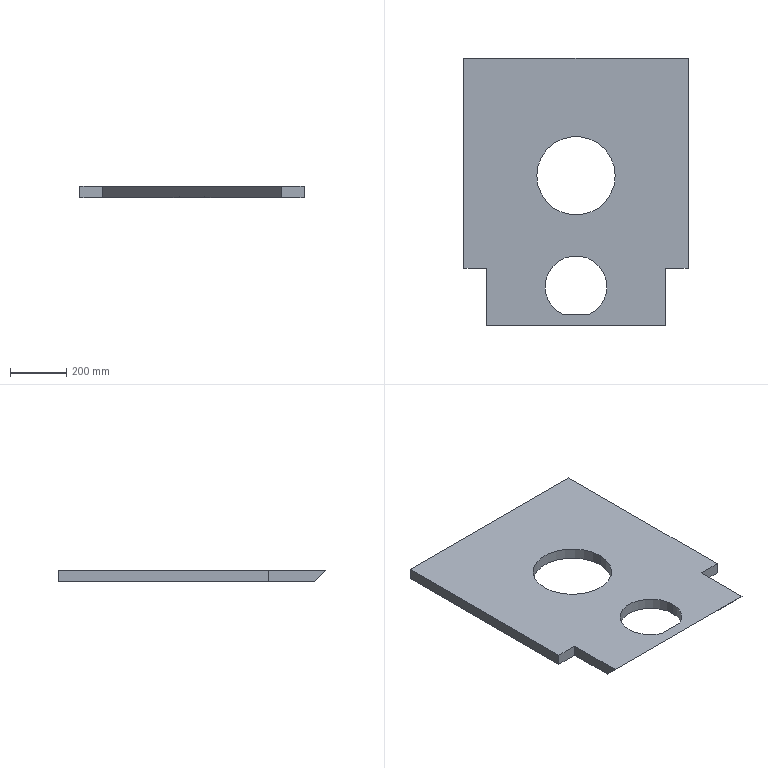Component | SolidWorks | JF21-80.1-1-3(_)-1-SOLID72-1 | 1 solid | 20 faces | box 800 x 956 x 40 mm | volume 24807837 mm3 | plane 11 | cylinder 7 | cone 2 | commonest cylinder face diameters 220 x3 8.5 x2 280 x2
STEP:
#1=CARTESIAN_POINT('',(0.,15.669,10.463));
#2=VERTEX_POINT('',#1);
#3=CARTESIAN_POINT('',(0.,15.669,10.797));
#4=VERTEX_POINT('',#3);
#5=CARTESIAN_POINT('',(0.,15.669,10.63));
#6=DIRECTION('',(0.,1.,0.));
#7=DIRECTION('',(0.,0.,1.));
#8=AXIS2_PLACEMENT_3D('',#5,#6,#7);
#9=CIRCLE('',#8,0.1673);
#10=EDGE_CURVE('',#2,#4,#9,.T.);
#11=ORIENTED_EDGE('',*,*,#10,.F.);
#12=CARTESIAN_POINT('',(0.,16.535,10.463));
#13=VERTEX_POINT('',#12);
#14=CARTESIAN_POINT('',(0.,16.535,10.463));
#15=DIRECTION('',(0.,1.,0.));
#16=VECTOR('',#15,39.37);
#17=LINE('',#14,#16);
#18=EDGE_CURVE('',#2,#13,#17,.T.);
#19=ORIENTED_EDGE('',*,*,#18,.T.);
#20=CARTESIAN_POINT('',(0.,16.535,10.797));
#21=VERTEX_POINT('',#20);
#22=CARTESIAN_POINT('',(0.,16.535,10.63));
#23=DIRECTION('',(0.,1.,0.));
#24=DIRECTION('',(0.,0.,1.));
#25=AXIS2_PLACEMENT_3D('',#22,#23,#24);
#26=CIRCLE('',#25,0.1673);
#27=EDGE_CURVE('',#13,#21,#26,.T.);
#28=ORIENTED_EDGE('',*,*,#27,.T.);
#29=CARTESIAN_POINT('',(0.,16.535,10.797));
#30=DIRECTION('',(0.,1.,0.));
#31=VECTOR('',#30,39.37);
#32=LINE('',#29,#31);
#33=EDGE_CURVE('',#4,#21,#32,.T.);
#34=ORIENTED_EDGE('',*,*,#33,.F.);
#35=EDGE_LOOP('',(#11,#19,#28,#34));
#36=FACE_OUTER_BOUND('',#35,.T.);
#37=CARTESIAN_POINT('',(0.,16.535,10.63));
#38=DIRECTION('',(0.,1.,0.));
#39=DIRECTION('',(0.,0.,-1.));
#40=AXIS2_PLACEMENT_3D('',#37,#38,#39);
#41=CYLINDRICAL_SURFACE('',#40,0.1673);
#42=ADVANCED_FACE('',(#36),#41,.F.);
#43=CARTESIAN_POINT('',(-0.,15.569,10.63));
#44=VERTEX_POINT('',#43);
#45=CARTESIAN_POINT('',(0.,15.669,10.797));
#46=DIRECTION('',(0.,0.515,0.8572));
#47=VECTOR('',#46,39.37);
#48=LINE('',#45,#47);
#49=EDGE_CURVE('',#44,#4,#48,.T.);
#50=ORIENTED_EDGE('',*,*,#49,.F.);
#51=CARTESIAN_POINT('',(0.,15.669,10.463));
#52=DIRECTION('',(0.,0.515,-0.8572));
#53=VECTOR('',#52,39.37);
#54=LINE('',#51,#53);
#55=EDGE_CURVE('',#44,#2,#54,.T.);
#56=ORIENTED_EDGE('',*,*,#55,.T.);
#57=ORIENTED_EDGE('',*,*,#10,.T.);
#58=EDGE_LOOP('',(#50,#56,#57));
#59=FACE_OUTER_BOUND('',#58,.T.);
#60=CARTESIAN_POINT('',(0.,15.669,10.63));
#61=DIRECTION('',(0.,1.,0.));
#62=DIRECTION('',(0.,0.,-1.));
#63=AXIS2_PLACEMENT_3D('',#60,#61,#62);
#64=CONICAL_SURFACE('',#63,0.1673,1.03);
#65=ADVANCED_FACE('',(#59),#64,.F.);
#66=CARTESIAN_POINT('',(1.804,-19.535,11.22));
#67=VERTEX_POINT('',#66);
#68=CARTESIAN_POINT('',(4.331,-15.598,11.22));
#69=VERTEX_POINT('',#68);
#70=CARTESIAN_POINT('',(0.,-15.598,11.22));
#71=DIRECTION('',(0.,0.,1.));
#72=DIRECTION('',(1.,0.,0.));
#73=AXIS2_PLACEMENT_3D('',#70,#71,#72);
#74=CIRCLE('',#73,4.331);
#75=EDGE_CURVE('',#67,#69,#74,.T.);
#76=ORIENTED_EDGE('',*,*,#75,.T.);
#77=CARTESIAN_POINT('',(4.331,-15.598,9.646));
#78=VERTEX_POINT('',#77);
#79=CARTESIAN_POINT('',(4.331,-15.598,11.22));
#80=DIRECTION('',(0.,0.,-1.));
#81=VECTOR('',#80,39.37);
#82=LINE('',#79,#81);
#83=EDGE_CURVE('',#69,#78,#82,.T.);
#84=ORIENTED_EDGE('',*,*,#83,.T.);
#85=CARTESIAN_POINT('',(1.82,-19.528,9.646));
#86=VERTEX_POINT('',#85);
#87=CARTESIAN_POINT('',(0.,-15.598,9.646));
#88=DIRECTION('',(0.,0.,1.));
#89=DIRECTION('',(1.,0.,0.));
#90=AXIS2_PLACEMENT_3D('',#87,#88,#89);
#91=CIRCLE('',#90,4.331);
#92=EDGE_CURVE('',#86,#78,#91,.T.);
#93=ORIENTED_EDGE('',*,*,#92,.F.);
#94=CARTESIAN_POINT('',(1.804,-19.535,9.653));
#95=VERTEX_POINT('',#94);
#96=CARTESIAN_POINT('',(1.82,-19.528,9.646));
#97=CARTESIAN_POINT('',(1.815,-19.53,9.648));
#98=CARTESIAN_POINT('',(1.81,-19.533,9.651));
#99=CARTESIAN_POINT('',(1.804,-19.535,9.653));
#100=(BOUNDED_CURVE()B_SPLINE_CURVE(3,(#96,#97,#98,#99),.UNSPECIFIED.,.F.,.T.)B_SPLINE_CURVE_WITH_KNOTS((4,4),(0.,1.),.UNSPECIFIED.)CURVE()GEOMETRIC_REPRESENTATION_ITEM()RATIONAL_B_SPLINE_CURVE((1.,1.,1.,1.))REPRESENTATION_ITEM(''));
#101=EDGE_CURVE('',#86,#95,#100,.T.);
#102=ORIENTED_EDGE('',*,*,#101,.T.);
#103=CARTESIAN_POINT('',(1.804,-19.535,11.22));
#104=DIRECTION('',(0.,0.,-1.));
#105=VECTOR('',#104,39.37);
#106=LINE('',#103,#105);
#107=EDGE_CURVE('',#67,#95,#106,.T.);
#108=ORIENTED_EDGE('',*,*,#107,.F.);
#109=EDGE_LOOP('',(#76,#84,#93,#102,#108));
#110=FACE_OUTER_BOUND('',#109,.T.);
#111=CARTESIAN_POINT('',(0.,-15.598,11.22));
#112=DIRECTION('',(0.,0.,-1.));
#113=DIRECTION('',(1.,0.,0.));
#114=AXIS2_PLACEMENT_3D('',#111,#112,#113);
#115=CYLINDRICAL_SURFACE('',#114,4.331);
#116=ADVANCED_FACE('',(#110),#115,.F.);
#117=ORIENTED_EDGE('',*,*,#83,.F.);
#118=CARTESIAN_POINT('',(-4.331,-15.598,11.22));
#119=VERTEX_POINT('',#118);
#120=CARTESIAN_POINT('',(0.,-15.598,11.22));
#121=DIRECTION('',(0.,0.,1.));
#122=DIRECTION('',(1.,0.,0.));
#123=AXIS2_PLACEMENT_3D('',#120,#121,#122);
#124=CIRCLE('',#123,4.331);
#125=EDGE_CURVE('',#69,#119,#124,.T.);
#126=ORIENTED_EDGE('',*,*,#125,.T.);
#127=CARTESIAN_POINT('',(-4.331,-15.598,9.646));
#128=VERTEX_POINT('',#127);
#129=CARTESIAN_POINT('',(-4.331,-15.598,11.22));
#130=DIRECTION('',(0.,0.,-1.));
#131=VECTOR('',#130,39.37);
#132=LINE('',#129,#131);
#133=EDGE_CURVE('',#119,#128,#132,.T.);
#134=ORIENTED_EDGE('',*,*,#133,.T.);
#135=CARTESIAN_POINT('',(0.,-15.598,9.646));
#136=DIRECTION('',(0.,0.,1.));
#137=DIRECTION('',(1.,0.,0.));
#138=AXIS2_PLACEMENT_3D('',#135,#136,#137);
#139=CIRCLE('',#138,4.331);
#140=EDGE_CURVE('',#78,#128,#139,.T.);
#141=ORIENTED_EDGE('',*,*,#140,.F.);
#142=EDGE_LOOP('',(#117,#126,#134,#141));
#143=FACE_OUTER_BOUND('',#142,.T.);
#144=CARTESIAN_POINT('',(0.,-15.598,11.22));
#145=DIRECTION('',(0.,0.,-1.));
#146=DIRECTION('',(1.,0.,0.));
#147=AXIS2_PLACEMENT_3D('',#144,#145,#146);
#148=CYLINDRICAL_SURFACE('',#147,4.331);
#149=ADVANCED_FACE('',(#143),#148,.F.);
#150=CARTESIAN_POINT('',(-5.512,0.,11.22));
#151=VERTEX_POINT('',#150);
#152=CARTESIAN_POINT('',(5.512,0.,11.22));
#153=VERTEX_POINT('',#152);
#154=CARTESIAN_POINT('',(0.,0.,11.22));
#155=DIRECTION('',(0.,0.,1.));
#156=DIRECTION('',(1.,0.,0.));
#157=AXIS2_PLACEMENT_3D('',#154,#155,#156);
#158=CIRCLE('',#157,5.512);
#159=EDGE_CURVE('',#151,#153,#158,.T.);
#160=ORIENTED_EDGE('',*,*,#159,.T.);
#161=CARTESIAN_POINT('',(5.512,0.,9.646));
#162=VERTEX_POINT('',#161);
#163=CARTESIAN_POINT('',(5.512,0.,11.22));
#164=DIRECTION('',(0.,0.,1.));
#165=VECTOR('',#164,39.37);
#166=LINE('',#163,#165);
#167=EDGE_CURVE('',#162,#153,#166,.T.);
#168=ORIENTED_EDGE('',*,*,#167,.F.);
#169=CARTESIAN_POINT('',(-5.512,0.,9.646));
#170=VERTEX_POINT('',#169);
#171=CARTESIAN_POINT('',(0.,0.,9.646));
#172=DIRECTION('',(0.,0.,1.));
#173=DIRECTION('',(1.,0.,0.));
#174=AXIS2_PLACEMENT_3D('',#171,#172,#173);
#175=CIRCLE('',#174,5.512);
#176=EDGE_CURVE('',#170,#162,#175,.T.);
#177=ORIENTED_EDGE('',*,*,#176,.F.);
#178=CARTESIAN_POINT('',(-5.512,0.,11.22));
#179=DIRECTION('',(0.,0.,1.));
#180=VECTOR('',#179,39.37);
#181=LINE('',#178,#180);
#182=EDGE_CURVE('',#170,#151,#181,.T.);
#183=ORIENTED_EDGE('',*,*,#182,.T.);
#184=EDGE_LOOP('',(#160,#168,#177,#183));
#185=FACE_OUTER_BOUND('',#184,.T.);
#186=CARTESIAN_POINT('',(0.,0.,11.22));
#187=DIRECTION('',(0.,0.,-1.));
#188=DIRECTION('',(1.,0.,0.));
#189=AXIS2_PLACEMENT_3D('',#186,#187,#188);
#190=CYLINDRICAL_SURFACE('',#189,5.512);
#191=ADVANCED_FACE('',(#185),#190,.F.);
#192=ORIENTED_EDGE('',*,*,#159,.F.);
#193=CARTESIAN_POINT('',(0.,0.,11.22));
#194=DIRECTION('',(0.,0.,1.));
#195=DIRECTION('',(1.,0.,0.));
#196=AXIS2_PLACEMENT_3D('',#193,#194,#195);
#197=CIRCLE('',#196,5.512);
#198=EDGE_CURVE('',#153,#151,#197,.T.);
#199=ORIENTED_EDGE('',*,*,#198,.F.);
#200=EDGE_LOOP('',(#192,#199));
#201=FACE_BOUND('',#200,.T.);
#202=CARTESIAN_POINT('',(15.748,-13.031,11.22));
#203=VERTEX_POINT('',#202);
#204=CARTESIAN_POINT('',(15.748,16.535,11.22));
#205=VERTEX_POINT('',#204);
#206=CARTESIAN_POINT('',(15.748,16.535,11.22));
#207=DIRECTION('',(0.,1.,0.));
#208=VECTOR('',#207,39.37);
#209=LINE('',#206,#208);
#210=EDGE_CURVE('',#203,#205,#209,.T.);
#211=ORIENTED_EDGE('',*,*,#210,.T.);
#212=CARTESIAN_POINT('',(-15.748,16.535,11.22));
#213=VERTEX_POINT('',#212);
#214=CARTESIAN_POINT('',(15.748,16.535,11.22));
#215=DIRECTION('',(-1.,-0.,0.));
#216=VECTOR('',#215,39.37);
#217=LINE('',#214,#216);
#218=EDGE_CURVE('',#205,#213,#217,.T.);
#219=ORIENTED_EDGE('',*,*,#218,.T.);
#220=CARTESIAN_POINT('',(-15.748,-13.031,11.22));
#221=VERTEX_POINT('',#220);
#222=CARTESIAN_POINT('',(-15.748,16.535,11.22));
#223=DIRECTION('',(0.,-1.,0.));
#224=VECTOR('',#223,39.37);
#225=LINE('',#222,#224);
#226=EDGE_CURVE('',#213,#221,#225,.T.);
#227=ORIENTED_EDGE('',*,*,#226,.T.);
#228=CARTESIAN_POINT('',(-12.598,-13.031,11.22));
#229=VERTEX_POINT('',#228);
#230=CARTESIAN_POINT('',(-12.598,-13.031,11.22));
#231=DIRECTION('',(1.,0.,0.));
#232=VECTOR('',#231,39.37);
#233=LINE('',#230,#232);
#234=EDGE_CURVE('',#221,#229,#233,.T.);
#235=ORIENTED_EDGE('',*,*,#234,.T.);
#236=CARTESIAN_POINT('',(-12.598,-21.102,11.22));
#237=VERTEX_POINT('',#236);
#238=CARTESIAN_POINT('',(-12.598,-13.031,11.22));
#239=DIRECTION('',(0.,-1.,0.));
#240=VECTOR('',#239,39.37);
#241=LINE('',#238,#240);
#242=EDGE_CURVE('',#229,#237,#241,.T.);
#243=ORIENTED_EDGE('',*,*,#242,.T.);
#244=CARTESIAN_POINT('',(12.598,-21.102,11.22));
#245=VERTEX_POINT('',#244);
#246=CARTESIAN_POINT('',(12.598,-21.102,11.22));
#247=DIRECTION('',(1.,0.,0.));
#248=VECTOR('',#247,39.37);
#249=LINE('',#246,#248);
#250=EDGE_CURVE('',#237,#245,#249,.T.);
#251=ORIENTED_EDGE('',*,*,#250,.T.);
#252=CARTESIAN_POINT('',(12.598,-13.031,11.22));
#253=VERTEX_POINT('',#252);
#254=CARTESIAN_POINT('',(12.598,-13.031,11.22));
#255=DIRECTION('',(0.,1.,0.));
#256=VECTOR('',#255,39.37);
#257=LINE('',#254,#256);
#258=EDGE_CURVE('',#245,#253,#257,.T.);
#259=ORIENTED_EDGE('',*,*,#258,.T.);
#260=CARTESIAN_POINT('',(12.598,-13.031,11.22));
#261=DIRECTION('',(1.,0.,0.));
#262=VECTOR('',#261,39.37);
#263=LINE('',#260,#262);
#264=EDGE_CURVE('',#253,#203,#263,.T.);
#265=ORIENTED_EDGE('',*,*,#264,.T.);
#266=EDGE_LOOP('',(#211,#219,#227,#235,#243,#251,#259,#265));
#267=FACE_OUTER_BOUND('',#266,.T.);
#268=CARTESIAN_POINT('',(-1.804,-19.535,11.22));
#269=VERTEX_POINT('',#268);
#270=CARTESIAN_POINT('',(-1.804,-19.535,11.22));
#271=DIRECTION('',(1.,-0.,0.));
#272=VECTOR('',#271,39.37);
#273=LINE('',#270,#272);
#274=EDGE_CURVE('',#269,#67,#273,.T.);
#275=ORIENTED_EDGE('',*,*,#274,.F.);
#276=CARTESIAN_POINT('',(0.,-15.598,11.22));
#277=DIRECTION('',(0.,0.,1.));
#278=DIRECTION('',(1.,0.,0.));
#279=AXIS2_PLACEMENT_3D('',#276,#277,#278);
#280=CIRCLE('',#279,4.331);
#281=EDGE_CURVE('',#119,#269,#280,.T.);
#282=ORIENTED_EDGE('',*,*,#281,.F.);
#283=ORIENTED_EDGE('',*,*,#125,.F.);
#284=ORIENTED_EDGE('',*,*,#75,.F.);
#285=EDGE_LOOP('',(#275,#282,#283,#284));
#286=FACE_BOUND('',#285,.T.);
#287=CARTESIAN_POINT('',(15.748,-13.031,11.22));
#288=DIRECTION('',(0.,0.,1.));
#289=DIRECTION('',(-1.,0.,0.));
#290=AXIS2_PLACEMENT_3D('',#287,#288,#289);
#291=PLANE('',#290);
#292=ADVANCED_FACE('',(#201,#267,#286),#291,.T.);
#293=ORIENTED_EDGE('',*,*,#176,.T.);
#294=CARTESIAN_POINT('',(0.,0.,9.646));
#295=DIRECTION('',(0.,0.,1.));
#296=DIRECTION('',(1.,0.,0.));
#297=AXIS2_PLACEMENT_3D('',#294,#295,#296);
#298=CIRCLE('',#297,5.512);
#299=EDGE_CURVE('',#162,#170,#298,.T.);
#300=ORIENTED_EDGE('',*,*,#299,.T.);
#301=EDGE_LOOP('',(#293,#300));
#302=FACE_BOUND('',#301,.T.);
#303=CARTESIAN_POINT('',(12.598,-19.528,9.646));
#304=VERTEX_POINT('',#303);
#305=CARTESIAN_POINT('',(12.598,-13.031,9.646));
#306=VERTEX_POINT('',#305);
#307=CARTESIAN_POINT('',(12.598,-13.031,9.646));
#308=DIRECTION('',(0.,1.,0.));
#309=VECTOR('',#308,39.37);
#310=LINE('',#307,#309);
#311=EDGE_CURVE('',#304,#306,#310,.T.);
#312=ORIENTED_EDGE('',*,*,#311,.F.);
#313=CARTESIAN_POINT('',(15.748,-19.528,9.646));
#314=DIRECTION('',(-1.,-0.,0.));
#315=VECTOR('',#314,39.37);
#316=LINE('',#313,#315);
#317=EDGE_CURVE('',#304,#86,#316,.T.);
#318=ORIENTED_EDGE('',*,*,#317,.T.);
#319=ORIENTED_EDGE('',*,*,#92,.T.);
#320=ORIENTED_EDGE('',*,*,#140,.T.);
#321=CARTESIAN_POINT('',(-1.82,-19.528,9.646));
#322=VERTEX_POINT('',#321);
#323=CARTESIAN_POINT('',(0.,-15.598,9.646));
#324=DIRECTION('',(0.,0.,1.));
#325=DIRECTION('',(1.,0.,0.));
#326=AXIS2_PLACEMENT_3D('',#323,#324,#325);
#327=CIRCLE('',#326,4.331);
#328=EDGE_CURVE('',#128,#322,#327,.T.);
#329=ORIENTED_EDGE('',*,*,#328,.T.);
#330=CARTESIAN_POINT('',(-12.598,-19.528,9.646));
#331=VERTEX_POINT('',#330);
#332=CARTESIAN_POINT('',(15.748,-19.528,9.646));
#333=DIRECTION('',(-1.,-0.,0.));
#334=VECTOR('',#333,39.37);
#335=LINE('',#332,#334);
#336=EDGE_CURVE('',#322,#331,#335,.T.);
#337=ORIENTED_EDGE('',*,*,#336,.T.);
#338=CARTESIAN_POINT('',(-12.598,-13.031,9.646));
#339=VERTEX_POINT('',#338);
#340=CARTESIAN_POINT('',(-12.598,-13.031,9.646));
#341=DIRECTION('',(0.,-1.,0.));
#342=VECTOR('',#341,39.37);
#343=LINE('',#340,#342);
#344=EDGE_CURVE('',#339,#331,#343,.T.);
#345=ORIENTED_EDGE('',*,*,#344,.F.);
#346=CARTESIAN_POINT('',(-15.748,-13.031,9.646));
#347=VERTEX_POINT('',#346);
#348=CARTESIAN_POINT('',(-12.598,-13.031,9.646));
#349=DIRECTION('',(1.,0.,0.));
#350=VECTOR('',#349,39.37);
#351=LINE('',#348,#350);
#352=EDGE_CURVE('',#347,#339,#351,.T.);
#353=ORIENTED_EDGE('',*,*,#352,.F.);
#354=CARTESIAN_POINT('',(-15.748,16.535,9.646));
#355=VERTEX_POINT('',#354);
#356=CARTESIAN_POINT('',(-15.748,16.535,9.646));
#357=DIRECTION('',(0.,-1.,0.));
#358=VECTOR('',#357,39.37);
#359=LINE('',#356,#358);
#360=EDGE_CURVE('',#355,#347,#359,.T.);
#361=ORIENTED_EDGE('',*,*,#360,.F.);
#362=CARTESIAN_POINT('',(15.748,16.535,9.646));
#363=VERTEX_POINT('',#362);
#364=CARTESIAN_POINT('',(15.748,16.535,9.646));
#365=DIRECTION('',(-1.,-0.,0.));
#366=VECTOR('',#365,39.37);
#367=LINE('',#364,#366);
#368=EDGE_CURVE('',#363,#355,#367,.T.);
#369=ORIENTED_EDGE('',*,*,#368,.F.);
#370=CARTESIAN_POINT('',(15.748,-13.031,9.646));
#371=VERTEX_POINT('',#370);
#372=CARTESIAN_POINT('',(15.748,16.535,9.646));
#373=DIRECTION('',(0.,1.,0.));
#374=VECTOR('',#373,39.37);
#375=LINE('',#372,#374);
#376=EDGE_CURVE('',#371,#363,#375,.T.);
#377=ORIENTED_EDGE('',*,*,#376,.F.);
#378=CARTESIAN_POINT('',(12.598,-13.031,9.646));
#379=DIRECTION('',(1.,0.,0.));
#380=VECTOR('',#379,39.37);
#381=LINE('',#378,#380);
#382=EDGE_CURVE('',#306,#371,#381,.T.);
#383=ORIENTED_EDGE('',*,*,#382,.F.);
#384=EDGE_LOOP('',(#312,#318,#319,#320,#329,#337,#345,#353,#361,#369,#377,#383));
#385=FACE_OUTER_BOUND('',#384,.T.);
#386=CARTESIAN_POINT('',(15.748,-13.031,9.646));
#387=DIRECTION('',(0.,0.,1.));
#388=DIRECTION('',(-1.,0.,0.));
#389=AXIS2_PLACEMENT_3D('',#386,#387,#388);
#390=PLANE('',#389);
#391=ADVANCED_FACE('',(#302,#385),#390,.F.);
#392=ORIENTED_EDGE('',*,*,#376,.T.);
#393=CARTESIAN_POINT('',(15.748,16.535,11.22));
#394=DIRECTION('',(0.,0.,-1.));
#395=VECTOR('',#394,39.37);
#396=LINE('',#393,#395);
#397=EDGE_CURVE('',#205,#363,#396,.T.);
#398=ORIENTED_EDGE('',*,*,#397,.F.);
#399=ORIENTED_EDGE('',*,*,#210,.F.);
#400=CARTESIAN_POINT('',(15.748,-13.031,11.22));
#401=DIRECTION('',(0.,0.,-1.));
#402=VECTOR('',#401,39.37);
#403=LINE('',#400,#402);
#404=EDGE_CURVE('',#203,#371,#403,.T.);
#405=ORIENTED_EDGE('',*,*,#404,.T.);
#406=EDGE_LOOP('',(#392,#398,#399,#405));
#407=FACE_OUTER_BOUND('',#406,.T.);
#408=CARTESIAN_POINT('',(15.748,16.535,11.22));
#409=DIRECTION('',(-1.,0.,0.));
#410=DIRECTION('',(0.,0.,-1.));
#411=AXIS2_PLACEMENT_3D('',#408,#409,#410);
#412=PLANE('',#411);
#413=ADVANCED_FACE('',(#407),#412,.F.);
#414=CARTESIAN_POINT('',(0.,16.535,10.63));
#415=DIRECTION('',(0.,1.,0.));
#416=DIRECTION('',(0.,0.,1.));
#417=AXIS2_PLACEMENT_3D('',#414,#415,#416);
#418=CIRCLE('',#417,0.1673);
#419=EDGE_CURVE('',#21,#13,#418,.T.);
#420=ORIENTED_EDGE('',*,*,#419,.F.);
#421=ORIENTED_EDGE('',*,*,#27,.F.);
#422=EDGE_LOOP('',(#420,#421));
#423=FACE_BOUND('',#422,.T.);
#424=ORIENTED_EDGE('',*,*,#368,.T.);
#425=CARTESIAN_POINT('',(-15.748,16.535,11.22));
#426=DIRECTION('',(0.,0.,-1.));
#427=VECTOR('',#426,39.37);
#428=LINE('',#425,#427);
#429=EDGE_CURVE('',#213,#355,#428,.T.);
#430=ORIENTED_EDGE('',*,*,#429,.F.);
#431=ORIENTED_EDGE('',*,*,#218,.F.);
#432=ORIENTED_EDGE('',*,*,#397,.T.);
#433=EDGE_LOOP('',(#424,#430,#431,#432));
#434=FACE_OUTER_BOUND('',#433,.T.);
#435=CARTESIAN_POINT('',(15.748,16.535,11.22));
#436=DIRECTION('',(0.,-1.,0.));
#437=DIRECTION('',(-1.,-0.,0.));
#438=AXIS2_PLACEMENT_3D('',#435,#436,#437);
#439=PLANE('',#438);
#440=ADVANCED_FACE('',(#423,#434),#439,.F.);
#441=ORIENTED_EDGE('',*,*,#360,.T.);
#442=CARTESIAN_POINT('',(-15.748,-13.031,11.22));
#443=DIRECTION('',(0.,0.,-1.));
#444=VECTOR('',#443,39.37);
#445=LINE('',#442,#444);
#446=EDGE_CURVE('',#221,#347,#445,.T.);
#447=ORIENTED_EDGE('',*,*,#446,.F.);
#448=ORIENTED_EDGE('',*,*,#226,.F.);
#449=ORIENTED_EDGE('',*,*,#429,.T.);
#450=EDGE_LOOP('',(#441,#447,#448,#449));
#451=FACE_OUTER_BOUND('',#450,.T.);
#452=CARTESIAN_POINT('',(-15.748,16.535,11.22));
#453=DIRECTION('',(1.,0.,0.));
#454=DIRECTION('',(0.,-1.,0.));
#455=AXIS2_PLACEMENT_3D('',#452,#453,#454);
#456=PLANE('',#455);
#457=ADVANCED_FACE('',(#451),#456,.F.);
#458=ORIENTED_EDGE('',*,*,#352,.T.);
#459=CARTESIAN_POINT('',(-12.598,-13.031,11.22));
#460=DIRECTION('',(0.,0.,-1.));
#461=VECTOR('',#460,39.37);
#462=LINE('',#459,#461);
#463=EDGE_CURVE('',#229,#339,#462,.T.);
#464=ORIENTED_EDGE('',*,*,#463,.F.);
#465=ORIENTED_EDGE('',*,*,#234,.F.);
#466=ORIENTED_EDGE('',*,*,#446,.T.);
#467=EDGE_LOOP('',(#458,#464,#465,#466));
#468=FACE_OUTER_BOUND('',#467,.T.);
#469=CARTESIAN_POINT('',(-12.598,-13.031,11.22));
#470=DIRECTION('',(0.,1.,0.));
#471=DIRECTION('',(0.,0.,-1.));
#472=AXIS2_PLACEMENT_3D('',#469,#470,#471);
#473=PLANE('',#472);
#474=ADVANCED_FACE('',(#468),#473,.F.);
#475=ORIENTED_EDGE('',*,*,#344,.T.);
#476=CARTESIAN_POINT('',(-12.598,-21.102,11.22));
#477=DIRECTION('',(0.,-0.7071,0.7071));
#478=VECTOR('',#477,39.37);
#479=LINE('',#476,#478);
#480=EDGE_CURVE('',#331,#237,#479,.T.);
#481=ORIENTED_EDGE('',*,*,#480,.T.);
#482=ORIENTED_EDGE('',*,*,#242,.F.);
#483=ORIENTED_EDGE('',*,*,#463,.T.);
#484=EDGE_LOOP('',(#475,#481,#482,#483));
#485=FACE_OUTER_BOUND('',#484,.T.);
#486=CARTESIAN_POINT('',(-12.598,-13.031,11.22));
#487=DIRECTION('',(1.,0.,0.));
#488=DIRECTION('',(0.,0.,1.));
#489=AXIS2_PLACEMENT_3D('',#486,#487,#488);
#490=PLANE('',#489);
#491=ADVANCED_FACE('',(#485),#490,.F.);
#492=ORIENTED_EDGE('',*,*,#258,.F.);
#493=CARTESIAN_POINT('',(12.598,-21.102,11.22));
#494=DIRECTION('',(0.,0.7071,-0.7071));
#495=VECTOR('',#494,39.37);
#496=LINE('',#493,#495);
#497=EDGE_CURVE('',#245,#304,#496,.T.);
#498=ORIENTED_EDGE('',*,*,#497,.T.);
#499=ORIENTED_EDGE('',*,*,#311,.T.);
#500=CARTESIAN_POINT('',(12.598,-13.031,11.22));
#501=DIRECTION('',(0.,0.,-1.));
#502=VECTOR('',#501,39.37);
#503=LINE('',#500,#502);
#504=EDGE_CURVE('',#253,#306,#503,.T.);
#505=ORIENTED_EDGE('',*,*,#504,.F.);
#506=EDGE_LOOP('',(#492,#498,#499,#505));
#507=FACE_OUTER_BOUND('',#506,.T.);
#508=CARTESIAN_POINT('',(12.598,-13.031,11.22));
#509=DIRECTION('',(-1.,0.,0.));
#510=DIRECTION('',(0.,0.,-1.));
#511=AXIS2_PLACEMENT_3D('',#508,#509,#510);
#512=PLANE('',#511);
#513=ADVANCED_FACE('',(#507),#512,.F.);
#514=ORIENTED_EDGE('',*,*,#382,.T.);
#515=ORIENTED_EDGE('',*,*,#404,.F.);
#516=ORIENTED_EDGE('',*,*,#264,.F.);
#517=ORIENTED_EDGE('',*,*,#504,.T.);
#518=EDGE_LOOP('',(#514,#515,#516,#517));
#519=FACE_OUTER_BOUND('',#518,.T.);
#520=CARTESIAN_POINT('',(12.598,-13.031,11.22));
#521=DIRECTION('',(0.,1.,0.));
#522=DIRECTION('',(0.,0.,-1.));
#523=AXIS2_PLACEMENT_3D('',#520,#521,#522);
#524=PLANE('',#523);
#525=ADVANCED_FACE('',(#519),#524,.F.);
#526=ORIENTED_EDGE('',*,*,#167,.T.);
#527=ORIENTED_EDGE('',*,*,#198,.T.);
#528=ORIENTED_EDGE('',*,*,#182,.F.);
#529=ORIENTED_EDGE('',*,*,#299,.F.);
#530=EDGE_LOOP('',(#526,#527,#528,#529));
#531=FACE_OUTER_BOUND('',#530,.T.);
#532=CARTESIAN_POINT('',(0.,0.,11.22));
#533=DIRECTION('',(0.,0.,-1.));
#534=DIRECTION('',(1.,0.,0.));
#535=AXIS2_PLACEMENT_3D('',#532,#533,#534);
#536=CYLINDRICAL_SURFACE('',#535,5.512);
#537=ADVANCED_FACE('',(#531),#536,.F.);
#538=ORIENTED_EDGE('',*,*,#133,.F.);
#539=ORIENTED_EDGE('',*,*,#281,.T.);
#540=CARTESIAN_POINT('',(-1.804,-19.535,9.653));
#541=VERTEX_POINT('',#540);
#542=CARTESIAN_POINT('',(-1.804,-19.535,11.22));
#543=DIRECTION('',(0.,0.,-1.));
#544=VECTOR('',#543,39.37);
#545=LINE('',#542,#544);
#546=EDGE_CURVE('',#269,#541,#545,.T.);
#547=ORIENTED_EDGE('',*,*,#546,.T.);
#548=CARTESIAN_POINT('',(-1.804,-19.535,9.653));
#549=CARTESIAN_POINT('',(-1.81,-19.533,9.651));
#550=CARTESIAN_POINT('',(-1.815,-19.53,9.648));
#551=CARTESIAN_POINT('',(-1.82,-19.528,9.646));
#552=(BOUNDED_CURVE()B_SPLINE_CURVE(3,(#548,#549,#550,#551),.UNSPECIFIED.,.F.,.T.)B_SPLINE_CURVE_WITH_KNOTS((4,4),(0.,1.),.UNSPECIFIED.)CURVE()GEOMETRIC_REPRESENTATION_ITEM()RATIONAL_B_SPLINE_CURVE((1.,1.,1.,1.))REPRESENTATION_ITEM(''));
#553=EDGE_CURVE('',#541,#322,#552,.T.);
#554=ORIENTED_EDGE('',*,*,#553,.T.);
#555=ORIENTED_EDGE('',*,*,#328,.F.);
#556=EDGE_LOOP('',(#538,#539,#547,#554,#555));
#557=FACE_OUTER_BOUND('',#556,.T.);
#558=CARTESIAN_POINT('',(0.,-15.598,11.22));
#559=DIRECTION('',(0.,0.,-1.));
#560=DIRECTION('',(1.,0.,0.));
#561=AXIS2_PLACEMENT_3D('',#558,#559,#560);
#562=CYLINDRICAL_SURFACE('',#561,4.331);
#563=ADVANCED_FACE('',(#557),#562,.F.);
#564=ORIENTED_EDGE('',*,*,#107,.T.);
#565=CARTESIAN_POINT('',(-1.804,-19.535,9.653));
#566=DIRECTION('',(-1.,0.,-0.));
#567=VECTOR('',#566,39.37);
#568=LINE('',#565,#567);
#569=EDGE_CURVE('',#95,#541,#568,.T.);
#570=ORIENTED_EDGE('',*,*,#569,.T.);
#571=ORIENTED_EDGE('',*,*,#546,.F.);
#572=ORIENTED_EDGE('',*,*,#274,.T.);
#573=EDGE_LOOP('',(#564,#570,#571,#572));
#574=FACE_OUTER_BOUND('',#573,.T.);
#575=CARTESIAN_POINT('',(-1.804,-19.535,11.22));
#576=DIRECTION('',(0.,1.,0.));
#577=DIRECTION('',(1.,-0.,0.));
#578=AXIS2_PLACEMENT_3D('',#575,#576,#577);
#579=PLANE('',#578);
#580=ADVANCED_FACE('',(#574),#579,.T.);
#581=ORIENTED_EDGE('',*,*,#101,.F.);
#582=ORIENTED_EDGE('',*,*,#317,.F.);
#583=ORIENTED_EDGE('',*,*,#497,.F.);
#584=ORIENTED_EDGE('',*,*,#250,.F.);
#585=ORIENTED_EDGE('',*,*,#480,.F.);
#586=ORIENTED_EDGE('',*,*,#336,.F.);
#587=ORIENTED_EDGE('',*,*,#553,.F.);
#588=ORIENTED_EDGE('',*,*,#569,.F.);
#589=EDGE_LOOP('',(#581,#582,#583,#584,#585,#586,#587,#588));
#590=FACE_OUTER_BOUND('',#589,.T.);
#591=CARTESIAN_POINT('',(12.598,-21.102,11.22));
#592=DIRECTION('',(-0.,0.7071,0.7071));
#593=DIRECTION('',(0.,0.7071,-0.7071));
#594=AXIS2_PLACEMENT_3D('',#591,#592,#593);
#595=PLANE('',#594);
#596=ADVANCED_FACE('',(#590),#595,.F.);
#597=ORIENTED_EDGE('',*,*,#55,.F.);
#598=ORIENTED_EDGE('',*,*,#49,.T.);
#599=CARTESIAN_POINT('',(0.,15.669,10.63));
#600=DIRECTION('',(0.,1.,0.));
#601=DIRECTION('',(0.,0.,1.));
#602=AXIS2_PLACEMENT_3D('',#599,#600,#601);
#603=CIRCLE('',#602,0.1673);
#604=EDGE_CURVE('',#4,#2,#603,.T.);
#605=ORIENTED_EDGE('',*,*,#604,.T.);
#606=EDGE_LOOP('',(#597,#598,#605));
#607=FACE_OUTER_BOUND('',#606,.T.);
#608=CARTESIAN_POINT('',(0.,15.669,10.63));
#609=DIRECTION('',(0.,1.,0.));
#610=DIRECTION('',(0.,0.,-1.));
#611=AXIS2_PLACEMENT_3D('',#608,#609,#610);
#612=CONICAL_SURFACE('',#611,0.1673,1.03);
#613=ADVANCED_FACE('',(#607),#612,.F.);
#614=ORIENTED_EDGE('',*,*,#18,.F.);
#615=ORIENTED_EDGE('',*,*,#604,.F.);
#616=ORIENTED_EDGE('',*,*,#33,.T.);
#617=ORIENTED_EDGE('',*,*,#419,.T.);
#618=EDGE_LOOP('',(#614,#615,#616,#617));
#619=FACE_OUTER_BOUND('',#618,.T.);
#620=CARTESIAN_POINT('',(0.,16.535,10.63));
#621=DIRECTION('',(0.,1.,0.));
#622=DIRECTION('',(0.,0.,-1.));
#623=AXIS2_PLACEMENT_3D('',#620,#621,#622);
#624=CYLINDRICAL_SURFACE('',#623,0.1673);
#625=ADVANCED_FACE('',(#619),#624,.F.);
#626=CLOSED_SHELL('',(#42,#65,#116,#149,#191,#292,#391,#413,#440,#457,#474,#491,#513,#525,#537,#563,#580,#596,#613,#625));
#627=MANIFOLD_SOLID_BREP('',#626);
#628=CARTESIAN_POINT('',(0.,0.,0.));
#629=DIRECTION('',(0.,0.,1.));
#630=DIRECTION('',(1.,0.,0.));
#631=AXIS2_PLACEMENT_3D('',#628,#629,#630);
#632=(LENGTH_UNIT()NAMED_UNIT(*)SI_UNIT($,.METRE.));
#633=LENGTH_MEASURE_WITH_UNIT(LENGTH_MEASURE(0.0254),#632);
#634=DIMENSIONAL_EXPONENTS(1.,0.,0.,0.,0.,0.,0.);
#635=(CONVERSION_BASED_UNIT('',#633)LENGTH_UNIT()NAMED_UNIT(#634));
#636=UNCERTAINTY_MEASURE_WITH_UNIT(LENGTH_MEASURE(0.00001),#635,'','');
#637=(NAMED_UNIT(*)PLANE_ANGLE_UNIT()SI_UNIT($,.RADIAN.));
#638=(NAMED_UNIT(*)SI_UNIT($,.STERADIAN.)SOLID_ANGLE_UNIT());
#639=(GEOMETRIC_REPRESENTATION_CONTEXT(3)GLOBAL_UNCERTAINTY_ASSIGNED_CONTEXT((#636))GLOBAL_UNIT_ASSIGNED_CONTEXT((#635,#637,#638))REPRESENTATION_CONTEXT('',''));
#640=ADVANCED_BREP_SHAPE_REPRESENTATION('',(#627,#631),#639);
#641=COLOUR_RGB('',0.7922,0.8196,0.9333);
#642=FILL_AREA_STYLE_COLOUR('',#641);
#643=FILL_AREA_STYLE('',(#642));
#644=SURFACE_STYLE_FILL_AREA(#643);
#645=SURFACE_SIDE_STYLE('',(#644));
#646=SURFACE_STYLE_USAGE(.BOTH.,#645);
#647=PRESENTATION_STYLE_ASSIGNMENT((#646));
#648=STYLED_ITEM('',(#647),#627);
#649=(LENGTH_UNIT()NAMED_UNIT(*)SI_UNIT($,.METRE.));
#650=LENGTH_MEASURE_WITH_UNIT(LENGTH_MEASURE(0.0254),#649);
#651=DIMENSIONAL_EXPONENTS(1.,0.,0.,0.,0.,0.,0.);
#652=(CONVERSION_BASED_UNIT('',#650)LENGTH_UNIT()NAMED_UNIT(#651));
#653=UNCERTAINTY_MEASURE_WITH_UNIT(LENGTH_MEASURE(0.00001),#652,'','');
#654=(NAMED_UNIT(*)PLANE_ANGLE_UNIT()SI_UNIT($,.RADIAN.));
#655=(NAMED_UNIT(*)SI_UNIT($,.STERADIAN.)SOLID_ANGLE_UNIT());
#656=(GEOMETRIC_REPRESENTATION_CONTEXT(3)GLOBAL_UNCERTAINTY_ASSIGNED_CONTEXT((#653))GLOBAL_UNIT_ASSIGNED_CONTEXT((#652,#654,#655))REPRESENTATION_CONTEXT('',''));
#657=MECHANICAL_DESIGN_GEOMETRIC_PRESENTATION_REPRESENTATION('',(#648),#656);
#658=PRESENTATION_LAYER_ASSIGNMENT('','',(#648));